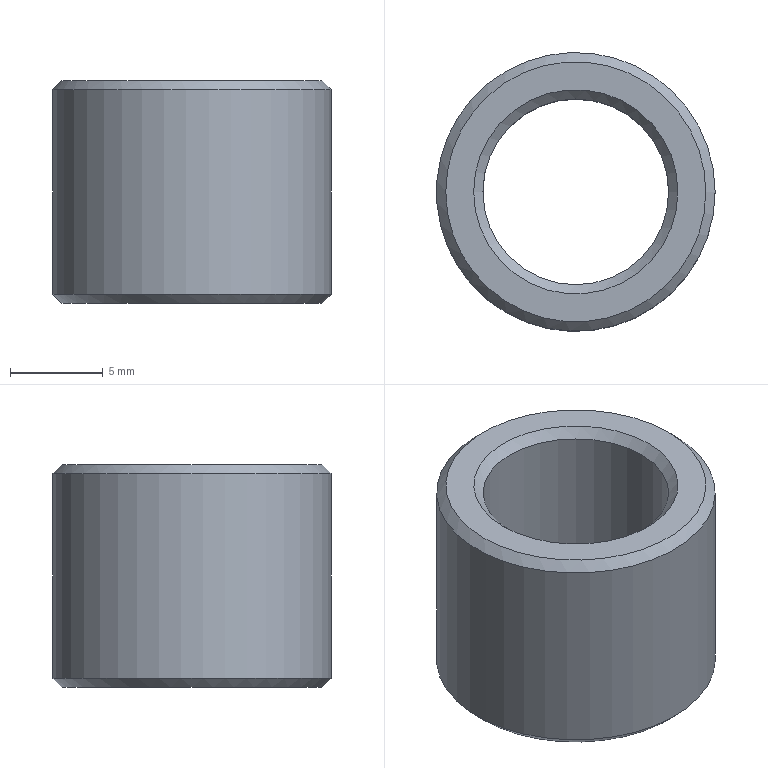Component | NX | BUSHING | 1 solid | 8 faces | box 15 x 15 x 12 mm | volume 1158 mm3 | cone 4 | cylinder 2 | plane 2 | commonest cylinder face diameters 15 x1 10 x1
STEP:
#1=CARTESIAN_POINT('',(0.,0.,0.));
#2=DIRECTION('',(0.,0.,1.));
#3=DIRECTION('',(1.,0.,0.));
#4=AXIS2_PLACEMENT_3D('',#1,#2,#3);
#5=CARTESIAN_POINT('',(19.5,100.638,-216.));
#6=VERTEX_POINT('',#5);
#7=CARTESIAN_POINT('',(12.,100.638,-216.));
#8=DIRECTION('',(0.,0.,1.));
#9=DIRECTION('',(1.,0.,0.));
#10=AXIS2_PLACEMENT_3D('',#7,#8,#9);
#11=CIRCLE('',#10,7.5);
#12=CARTESIAN_POINT('',(12.,100.638,-204.5));
#13=DIRECTION('',(0.,0.,-1.));
#14=DIRECTION('',(-1.,0.,0.));
#15=AXIS2_PLACEMENT_3D('',#12,#13,#14);
#16=CYLINDRICAL_SURFACE('',#15,7.5);
#17=CARTESIAN_POINT('',(9.425,11.5));
#18=DIRECTION('',(-1.,0.));
#19=VECTOR('',#18,1.);
#20=LINE('',#17,#19);
#21=(GEOMETRIC_REPRESENTATION_CONTEXT(2)PARAMETRIC_REPRESENTATION_CONTEXT()REPRESENTATION_CONTEXT('',''));
#22=DEFINITIONAL_REPRESENTATION('',(#20),#21);
#23=PCURVE('',#16,#22);
#24=CARTESIAN_POINT('',(12.,100.638,-216.));
#25=DIRECTION('',(0.,0.,1.));
#26=DIRECTION('',(1.,0.,0.));
#27=AXIS2_PLACEMENT_3D('',#24,#25,#26);
#28=CONICAL_SURFACE('',#27,7.5,0.7854);
#29=CARTESIAN_POINT('',(0.,0.));
#30=DIRECTION('',(1.,0.));
#31=VECTOR('',#30,1.);
#32=LINE('',#29,#31);
#33=(GEOMETRIC_REPRESENTATION_CONTEXT(2)PARAMETRIC_REPRESENTATION_CONTEXT()REPRESENTATION_CONTEXT('',''));
#34=DEFINITIONAL_REPRESENTATION('',(#32),#33);
#35=PCURVE('',#28,#34);
#36=SURFACE_CURVE('',#11,(#23,#35),.PCURVE_S1.);
#37=EDGE_CURVE('',#6,#6,#36,.T.);
#38=ORIENTED_EDGE('',*,*,#37,.T.);
#39=CARTESIAN_POINT('',(19.5,100.638,-205.));
#40=VERTEX_POINT('',#39);
#41=CARTESIAN_POINT('',(19.5,100.638,-205.));
#42=CARTESIAN_POINT('',(19.5,100.638,-216.));
#43=B_SPLINE_CURVE_WITH_KNOTS('',1,(#41,#42),.UNSPECIFIED.,.F.,.F.,(2,2),(0.5,11.5),.PIECEWISE_BEZIER_KNOTS.);
#44=CARTESIAN_POINT('',(3.142,0.));
#45=DIRECTION('',(0.,1.));
#46=VECTOR('',#45,1.);
#47=LINE('',#44,#46);
#48=(GEOMETRIC_REPRESENTATION_CONTEXT(2)PARAMETRIC_REPRESENTATION_CONTEXT()REPRESENTATION_CONTEXT('',''));
#49=DEFINITIONAL_REPRESENTATION('',(#47),#48);
#50=PCURVE('',#16,#49);
#51=CARTESIAN_POINT('',(9.425,0.));
#52=DIRECTION('',(0.,1.));
#53=VECTOR('',#52,1.);
#54=LINE('',#51,#53);
#55=(GEOMETRIC_REPRESENTATION_CONTEXT(2)PARAMETRIC_REPRESENTATION_CONTEXT()REPRESENTATION_CONTEXT('',''));
#56=DEFINITIONAL_REPRESENTATION('',(#54),#55);
#57=PCURVE('',#16,#56);
#58=SEAM_CURVE('',#43,(#50,#57),.PCURVE_S1.);
#59=EDGE_CURVE('',#40,#6,#58,.T.);
#60=ORIENTED_EDGE('',*,*,#59,.F.);
#61=CARTESIAN_POINT('',(12.,100.638,-205.));
#62=DIRECTION('',(0.,0.,-1.));
#63=DIRECTION('',(1.,0.,0.));
#64=AXIS2_PLACEMENT_3D('',#61,#62,#63);
#65=CIRCLE('',#64,7.5);
#66=CARTESIAN_POINT('',(3.142,0.5));
#67=DIRECTION('',(1.,0.));
#68=VECTOR('',#67,1.);
#69=LINE('',#66,#68);
#70=(GEOMETRIC_REPRESENTATION_CONTEXT(2)PARAMETRIC_REPRESENTATION_CONTEXT()REPRESENTATION_CONTEXT('',''));
#71=DEFINITIONAL_REPRESENTATION('',(#69),#70);
#72=PCURVE('',#16,#71);
#73=CARTESIAN_POINT('',(12.,100.638,-204.5));
#74=DIRECTION('',(0.,0.,-1.));
#75=DIRECTION('',(-1.,0.,0.));
#76=AXIS2_PLACEMENT_3D('',#73,#74,#75);
#77=CONICAL_SURFACE('',#76,7.,0.7854);
#78=CARTESIAN_POINT('',(3.142,0.5));
#79=DIRECTION('',(1.,0.));
#80=VECTOR('',#79,1.);
#81=LINE('',#78,#80);
#82=(GEOMETRIC_REPRESENTATION_CONTEXT(2)PARAMETRIC_REPRESENTATION_CONTEXT()REPRESENTATION_CONTEXT('',''));
#83=DEFINITIONAL_REPRESENTATION('',(#81),#82);
#84=PCURVE('',#77,#83);
#85=SURFACE_CURVE('',#65,(#72,#84),.PCURVE_S1.);
#86=EDGE_CURVE('',#40,#40,#85,.T.);
#87=ORIENTED_EDGE('',*,*,#86,.T.);
#88=ORIENTED_EDGE('',*,*,#59,.T.);
#89=EDGE_LOOP('',(#38,#60,#87,#88));
#90=FACE_BOUND('',#89,.T.);
#91=ADVANCED_FACE('',(#90),#16,.T.);
#92=CARTESIAN_POINT('',(17.,100.638,-216.));
#93=VERTEX_POINT('',#92);
#94=CARTESIAN_POINT('',(12.,100.638,-216.));
#95=DIRECTION('',(0.,0.,-1.));
#96=DIRECTION('',(1.,0.,0.));
#97=AXIS2_PLACEMENT_3D('',#94,#95,#96);
#98=CIRCLE('',#97,5.);
#99=CARTESIAN_POINT('',(12.,100.638,-204.5));
#100=DIRECTION('',(0.,0.,-1.));
#101=DIRECTION('',(-1.,0.,0.));
#102=AXIS2_PLACEMENT_3D('',#99,#100,#101);
#103=CYLINDRICAL_SURFACE('',#102,5.);
#104=CARTESIAN_POINT('',(3.142,11.5));
#105=DIRECTION('',(1.,0.));
#106=VECTOR('',#105,1.);
#107=LINE('',#104,#106);
#108=(GEOMETRIC_REPRESENTATION_CONTEXT(2)PARAMETRIC_REPRESENTATION_CONTEXT()REPRESENTATION_CONTEXT('',''));
#109=DEFINITIONAL_REPRESENTATION('',(#107),#108);
#110=PCURVE('',#103,#109);
#111=CARTESIAN_POINT('',(12.,100.638,-216.5));
#112=DIRECTION('',(0.,0.,-1.));
#113=DIRECTION('',(-1.,0.,0.));
#114=AXIS2_PLACEMENT_3D('',#111,#112,#113);
#115=CONICAL_SURFACE('',#114,5.5,0.7854);
#116=CARTESIAN_POINT('',(3.142,-0.5));
#117=DIRECTION('',(1.,0.));
#118=VECTOR('',#117,1.);
#119=LINE('',#116,#118);
#120=(GEOMETRIC_REPRESENTATION_CONTEXT(2)PARAMETRIC_REPRESENTATION_CONTEXT()REPRESENTATION_CONTEXT('',''));
#121=DEFINITIONAL_REPRESENTATION('',(#119),#120);
#122=PCURVE('',#115,#121);
#123=SURFACE_CURVE('',#98,(#110,#122),.PCURVE_S1.);
#124=EDGE_CURVE('',#93,#93,#123,.T.);
#125=ORIENTED_EDGE('',*,*,#124,.F.);
#126=CARTESIAN_POINT('',(17.,100.638,-205.));
#127=VERTEX_POINT('',#126);
#128=CARTESIAN_POINT('',(17.,100.638,-205.));
#129=CARTESIAN_POINT('',(17.,100.638,-216.));
#130=B_SPLINE_CURVE_WITH_KNOTS('',1,(#128,#129),.UNSPECIFIED.,.F.,.F.,(2,2),(0.5,11.5),.PIECEWISE_BEZIER_KNOTS.);
#131=CARTESIAN_POINT('',(3.142,0.));
#132=DIRECTION('',(0.,1.));
#133=VECTOR('',#132,1.);
#134=LINE('',#131,#133);
#135=(GEOMETRIC_REPRESENTATION_CONTEXT(2)PARAMETRIC_REPRESENTATION_CONTEXT()REPRESENTATION_CONTEXT('',''));
#136=DEFINITIONAL_REPRESENTATION('',(#134),#135);
#137=PCURVE('',#103,#136);
#138=CARTESIAN_POINT('',(9.425,0.));
#139=DIRECTION('',(0.,1.));
#140=VECTOR('',#139,1.);
#141=LINE('',#138,#140);
#142=(GEOMETRIC_REPRESENTATION_CONTEXT(2)PARAMETRIC_REPRESENTATION_CONTEXT()REPRESENTATION_CONTEXT('',''));
#143=DEFINITIONAL_REPRESENTATION('',(#141),#142);
#144=PCURVE('',#103,#143);
#145=SEAM_CURVE('',#130,(#137,#144),.PCURVE_S1.);
#146=EDGE_CURVE('',#127,#93,#145,.T.);
#147=ORIENTED_EDGE('',*,*,#146,.F.);
#148=CARTESIAN_POINT('',(12.,100.638,-205.));
#149=DIRECTION('',(0.,0.,1.));
#150=DIRECTION('',(1.,0.,0.));
#151=AXIS2_PLACEMENT_3D('',#148,#149,#150);
#152=CIRCLE('',#151,5.);
#153=CARTESIAN_POINT('',(9.425,0.5));
#154=DIRECTION('',(-1.,0.));
#155=VECTOR('',#154,1.);
#156=LINE('',#153,#155);
#157=(GEOMETRIC_REPRESENTATION_CONTEXT(2)PARAMETRIC_REPRESENTATION_CONTEXT()REPRESENTATION_CONTEXT('',''));
#158=DEFINITIONAL_REPRESENTATION('',(#156),#157);
#159=PCURVE('',#103,#158);
#160=CARTESIAN_POINT('',(12.,100.638,-205.));
#161=DIRECTION('',(0.,0.,1.));
#162=DIRECTION('',(1.,0.,0.));
#163=AXIS2_PLACEMENT_3D('',#160,#161,#162);
#164=CONICAL_SURFACE('',#163,5.,0.7854);
#165=CARTESIAN_POINT('',(0.,0.));
#166=DIRECTION('',(1.,0.));
#167=VECTOR('',#166,1.);
#168=LINE('',#165,#167);
#169=(GEOMETRIC_REPRESENTATION_CONTEXT(2)PARAMETRIC_REPRESENTATION_CONTEXT()REPRESENTATION_CONTEXT('',''));
#170=DEFINITIONAL_REPRESENTATION('',(#168),#169);
#171=PCURVE('',#164,#170);
#172=SURFACE_CURVE('',#152,(#159,#171),.PCURVE_S1.);
#173=EDGE_CURVE('',#127,#127,#172,.T.);
#174=ORIENTED_EDGE('',*,*,#173,.F.);
#175=ORIENTED_EDGE('',*,*,#146,.T.);
#176=EDGE_LOOP('',(#125,#147,#174,#175));
#177=FACE_BOUND('',#176,.F.);
#178=ADVANCED_FACE('',(#177),#103,.F.);
#179=CARTESIAN_POINT('',(17.5,100.638,-204.5));
#180=VERTEX_POINT('',#179);
#181=CARTESIAN_POINT('',(12.,100.638,-204.5));
#182=DIRECTION('',(0.,0.,-1.));
#183=DIRECTION('',(1.,0.,0.));
#184=AXIS2_PLACEMENT_3D('',#181,#182,#183);
#185=CIRCLE('',#184,5.5);
#186=CARTESIAN_POINT('',(12.,100.638,-204.5));
#187=DIRECTION('',(0.,0.,1.));
#188=DIRECTION('',(1.,0.,0.));
#189=AXIS2_PLACEMENT_3D('',#186,#187,#188);
#190=PLANE('',#189);
#191=CARTESIAN_POINT('',(5.5,0.));
#192=CARTESIAN_POINT('',(5.5,-9.526));
#193=CARTESIAN_POINT('',(-2.75,-4.763));
#194=CARTESIAN_POINT('',(-11.,-0.));
#195=CARTESIAN_POINT('',(-2.75,4.763));
#196=CARTESIAN_POINT('',(5.5,9.526));
#197=CARTESIAN_POINT('',(5.5,0.));
#198=(BOUNDED_CURVE()B_SPLINE_CURVE(2,(#191,#192,#193,#194,#195,#196,#197),.UNSPECIFIED.,.T.,.F.)B_SPLINE_CURVE_WITH_KNOTS((1,2,2,2,2,1),(-2.094,0.,2.094,4.189,6.283,8.378),.UNSPECIFIED.)CURVE()GEOMETRIC_REPRESENTATION_ITEM()RATIONAL_B_SPLINE_CURVE((1.,0.5,1.,0.5,1.,0.5,1.))REPRESENTATION_ITEM(''));
#199=(GEOMETRIC_REPRESENTATION_CONTEXT(2)PARAMETRIC_REPRESENTATION_CONTEXT()REPRESENTATION_CONTEXT('',''));
#200=DEFINITIONAL_REPRESENTATION('',(#198),#199);
#201=PCURVE('',#190,#200);
#202=CARTESIAN_POINT('',(6.283,0.5));
#203=DIRECTION('',(-1.,0.));
#204=VECTOR('',#203,1.);
#205=LINE('',#202,#204);
#206=(GEOMETRIC_REPRESENTATION_CONTEXT(2)PARAMETRIC_REPRESENTATION_CONTEXT()REPRESENTATION_CONTEXT('',''));
#207=DEFINITIONAL_REPRESENTATION('',(#205),#206);
#208=PCURVE('',#164,#207);
#209=SURFACE_CURVE('',#185,(#201,#208),.PCURVE_S1.);
#210=EDGE_CURVE('',#180,#180,#209,.T.);
#211=ORIENTED_EDGE('',*,*,#210,.T.);
#212=EDGE_LOOP('',(#211));
#213=FACE_BOUND('',#212,.T.);
#214=CARTESIAN_POINT('',(19.,100.638,-204.5));
#215=VERTEX_POINT('',#214);
#216=CARTESIAN_POINT('',(12.,100.638,-204.5));
#217=DIRECTION('',(0.,0.,1.));
#218=DIRECTION('',(1.,0.,0.));
#219=AXIS2_PLACEMENT_3D('',#216,#217,#218);
#220=CIRCLE('',#219,7.);
#221=CARTESIAN_POINT('',(0.,0.));
#222=DIRECTION('',(1.,0.));
#223=AXIS2_PLACEMENT_2D('',#221,#222);
#224=CIRCLE('',#223,7.);
#225=(GEOMETRIC_REPRESENTATION_CONTEXT(2)PARAMETRIC_REPRESENTATION_CONTEXT()REPRESENTATION_CONTEXT('',''));
#226=DEFINITIONAL_REPRESENTATION('',(#224),#225);
#227=PCURVE('',#190,#226);
#228=CARTESIAN_POINT('',(9.425,0.));
#229=DIRECTION('',(-1.,0.));
#230=VECTOR('',#229,1.);
#231=LINE('',#228,#230);
#232=(GEOMETRIC_REPRESENTATION_CONTEXT(2)PARAMETRIC_REPRESENTATION_CONTEXT()REPRESENTATION_CONTEXT('',''));
#233=DEFINITIONAL_REPRESENTATION('',(#231),#232);
#234=PCURVE('',#77,#233);
#235=SURFACE_CURVE('',#220,(#227,#234),.PCURVE_S1.);
#236=EDGE_CURVE('',#215,#215,#235,.T.);
#237=ORIENTED_EDGE('',*,*,#236,.T.);
#238=EDGE_LOOP('',(#237));
#239=FACE_BOUND('',#238,.T.);
#240=ADVANCED_FACE('',(#213,#239),#190,.T.);
#241=CARTESIAN_POINT('',(17.5,100.638,-216.5));
#242=VERTEX_POINT('',#241);
#243=CARTESIAN_POINT('',(12.,100.638,-216.5));
#244=DIRECTION('',(0.,0.,1.));
#245=DIRECTION('',(1.,0.,0.));
#246=AXIS2_PLACEMENT_3D('',#243,#244,#245);
#247=CIRCLE('',#246,5.5);
#248=CARTESIAN_POINT('',(12.,100.638,-216.5));
#249=DIRECTION('',(0.,0.,1.));
#250=DIRECTION('',(1.,0.,0.));
#251=AXIS2_PLACEMENT_3D('',#248,#249,#250);
#252=PLANE('',#251);
#253=CARTESIAN_POINT('',(0.,0.));
#254=DIRECTION('',(1.,0.));
#255=AXIS2_PLACEMENT_2D('',#253,#254);
#256=CIRCLE('',#255,5.5);
#257=(GEOMETRIC_REPRESENTATION_CONTEXT(2)PARAMETRIC_REPRESENTATION_CONTEXT()REPRESENTATION_CONTEXT('',''));
#258=DEFINITIONAL_REPRESENTATION('',(#256),#257);
#259=PCURVE('',#252,#258);
#260=CARTESIAN_POINT('',(9.425,0.));
#261=DIRECTION('',(-1.,0.));
#262=VECTOR('',#261,1.);
#263=LINE('',#260,#262);
#264=(GEOMETRIC_REPRESENTATION_CONTEXT(2)PARAMETRIC_REPRESENTATION_CONTEXT()REPRESENTATION_CONTEXT('',''));
#265=DEFINITIONAL_REPRESENTATION('',(#263),#264);
#266=PCURVE('',#115,#265);
#267=SURFACE_CURVE('',#247,(#259,#266),.PCURVE_S1.);
#268=EDGE_CURVE('',#242,#242,#267,.T.);
#269=ORIENTED_EDGE('',*,*,#268,.T.);
#270=EDGE_LOOP('',(#269));
#271=FACE_BOUND('',#270,.T.);
#272=CARTESIAN_POINT('',(19.,100.638,-216.5));
#273=VERTEX_POINT('',#272);
#274=CARTESIAN_POINT('',(12.,100.638,-216.5));
#275=DIRECTION('',(0.,0.,-1.));
#276=DIRECTION('',(1.,0.,0.));
#277=AXIS2_PLACEMENT_3D('',#274,#275,#276);
#278=CIRCLE('',#277,7.);
#279=CARTESIAN_POINT('',(7.,0.));
#280=CARTESIAN_POINT('',(7.,-12.124));
#281=CARTESIAN_POINT('',(-3.5,-6.062));
#282=CARTESIAN_POINT('',(-14.,-0.));
#283=CARTESIAN_POINT('',(-3.5,6.062));
#284=CARTESIAN_POINT('',(7.,12.124));
#285=CARTESIAN_POINT('',(7.,0.));
#286=(BOUNDED_CURVE()B_SPLINE_CURVE(2,(#279,#280,#281,#282,#283,#284,#285),.UNSPECIFIED.,.T.,.F.)B_SPLINE_CURVE_WITH_KNOTS((1,2,2,2,2,1),(-2.094,0.,2.094,4.189,6.283,8.378),.UNSPECIFIED.)CURVE()GEOMETRIC_REPRESENTATION_ITEM()RATIONAL_B_SPLINE_CURVE((1.,0.5,1.,0.5,1.,0.5,1.))REPRESENTATION_ITEM(''));
#287=(GEOMETRIC_REPRESENTATION_CONTEXT(2)PARAMETRIC_REPRESENTATION_CONTEXT()REPRESENTATION_CONTEXT('',''));
#288=DEFINITIONAL_REPRESENTATION('',(#286),#287);
#289=PCURVE('',#252,#288);
#290=CARTESIAN_POINT('',(6.283,-0.5));
#291=DIRECTION('',(-1.,0.));
#292=VECTOR('',#291,1.);
#293=LINE('',#290,#292);
#294=(GEOMETRIC_REPRESENTATION_CONTEXT(2)PARAMETRIC_REPRESENTATION_CONTEXT()REPRESENTATION_CONTEXT('',''));
#295=DEFINITIONAL_REPRESENTATION('',(#293),#294);
#296=PCURVE('',#28,#295);
#297=SURFACE_CURVE('',#278,(#289,#296),.PCURVE_S1.);
#298=EDGE_CURVE('',#273,#273,#297,.T.);
#299=ORIENTED_EDGE('',*,*,#298,.T.);
#300=EDGE_LOOP('',(#299));
#301=FACE_BOUND('',#300,.T.);
#302=ADVANCED_FACE('',(#271,#301),#252,.F.);
#303=ORIENTED_EDGE('',*,*,#124,.T.);
#304=CARTESIAN_POINT('',(17.,100.638,-216.));
#305=CARTESIAN_POINT('',(17.5,100.638,-216.5));
#306=B_SPLINE_CURVE_WITH_KNOTS('',1,(#304,#305),.UNSPECIFIED.,.F.,.F.,(2,2),(-0.7071,0.),.PIECEWISE_BEZIER_KNOTS.);
#307=CARTESIAN_POINT('',(9.425,0.));
#308=DIRECTION('',(0.,1.));
#309=VECTOR('',#308,1.);
#310=LINE('',#307,#309);
#311=(GEOMETRIC_REPRESENTATION_CONTEXT(2)PARAMETRIC_REPRESENTATION_CONTEXT()REPRESENTATION_CONTEXT('',''));
#312=DEFINITIONAL_REPRESENTATION('',(#310),#311);
#313=PCURVE('',#115,#312);
#314=CARTESIAN_POINT('',(3.142,0.));
#315=DIRECTION('',(0.,1.));
#316=VECTOR('',#315,1.);
#317=LINE('',#314,#316);
#318=(GEOMETRIC_REPRESENTATION_CONTEXT(2)PARAMETRIC_REPRESENTATION_CONTEXT()REPRESENTATION_CONTEXT('',''));
#319=DEFINITIONAL_REPRESENTATION('',(#317),#318);
#320=PCURVE('',#115,#319);
#321=SEAM_CURVE('',#306,(#313,#320),.PCURVE_S1.);
#322=EDGE_CURVE('',#93,#242,#321,.T.);
#323=ORIENTED_EDGE('',*,*,#322,.T.);
#324=ORIENTED_EDGE('',*,*,#268,.T.);
#325=ORIENTED_EDGE('',*,*,#322,.F.);
#326=EDGE_LOOP('',(#303,#323,#324,#325));
#327=FACE_BOUND('',#326,.F.);
#328=ADVANCED_FACE('',(#327),#115,.F.);
#329=ORIENTED_EDGE('',*,*,#298,.F.);
#330=CARTESIAN_POINT('',(19.,100.638,-216.5));
#331=CARTESIAN_POINT('',(19.5,100.638,-216.));
#332=B_SPLINE_CURVE_WITH_KNOTS('',1,(#330,#331),.UNSPECIFIED.,.F.,.F.,(2,2),(-0.7071,0.),.PIECEWISE_BEZIER_KNOTS.);
#333=CARTESIAN_POINT('',(6.283,0.));
#334=DIRECTION('',(0.,1.));
#335=VECTOR('',#334,1.);
#336=LINE('',#333,#335);
#337=(GEOMETRIC_REPRESENTATION_CONTEXT(2)PARAMETRIC_REPRESENTATION_CONTEXT()REPRESENTATION_CONTEXT('',''));
#338=DEFINITIONAL_REPRESENTATION('',(#336),#337);
#339=PCURVE('',#28,#338);
#340=CARTESIAN_POINT('',(0.,0.));
#341=DIRECTION('',(0.,1.));
#342=VECTOR('',#341,1.);
#343=LINE('',#340,#342);
#344=(GEOMETRIC_REPRESENTATION_CONTEXT(2)PARAMETRIC_REPRESENTATION_CONTEXT()REPRESENTATION_CONTEXT('',''));
#345=DEFINITIONAL_REPRESENTATION('',(#343),#344);
#346=PCURVE('',#28,#345);
#347=SEAM_CURVE('',#332,(#339,#346),.PCURVE_S1.);
#348=EDGE_CURVE('',#273,#6,#347,.T.);
#349=ORIENTED_EDGE('',*,*,#348,.T.);
#350=ORIENTED_EDGE('',*,*,#37,.F.);
#351=ORIENTED_EDGE('',*,*,#348,.F.);
#352=EDGE_LOOP('',(#329,#349,#350,#351));
#353=FACE_BOUND('',#352,.T.);
#354=ADVANCED_FACE('',(#353),#28,.T.);
#355=ORIENTED_EDGE('',*,*,#210,.T.);
#356=CARTESIAN_POINT('',(17.,100.638,-205.));
#357=CARTESIAN_POINT('',(17.5,100.638,-204.5));
#358=B_SPLINE_CURVE_WITH_KNOTS('',1,(#356,#357),.UNSPECIFIED.,.F.,.F.,(2,2),(0.,0.7071),.PIECEWISE_BEZIER_KNOTS.);
#359=CARTESIAN_POINT('',(0.,0.));
#360=DIRECTION('',(0.,1.));
#361=VECTOR('',#360,1.);
#362=LINE('',#359,#361);
#363=(GEOMETRIC_REPRESENTATION_CONTEXT(2)PARAMETRIC_REPRESENTATION_CONTEXT()REPRESENTATION_CONTEXT('',''));
#364=DEFINITIONAL_REPRESENTATION('',(#362),#363);
#365=PCURVE('',#164,#364);
#366=CARTESIAN_POINT('',(6.283,0.));
#367=DIRECTION('',(0.,1.));
#368=VECTOR('',#367,1.);
#369=LINE('',#366,#368);
#370=(GEOMETRIC_REPRESENTATION_CONTEXT(2)PARAMETRIC_REPRESENTATION_CONTEXT()REPRESENTATION_CONTEXT('',''));
#371=DEFINITIONAL_REPRESENTATION('',(#369),#370);
#372=PCURVE('',#164,#371);
#373=SEAM_CURVE('',#358,(#365,#372),.PCURVE_S1.);
#374=EDGE_CURVE('',#127,#180,#373,.T.);
#375=ORIENTED_EDGE('',*,*,#374,.F.);
#376=ORIENTED_EDGE('',*,*,#173,.T.);
#377=ORIENTED_EDGE('',*,*,#374,.T.);
#378=EDGE_LOOP('',(#355,#375,#376,#377));
#379=FACE_BOUND('',#378,.F.);
#380=ADVANCED_FACE('',(#379),#164,.F.);
#381=ORIENTED_EDGE('',*,*,#86,.F.);
#382=CARTESIAN_POINT('',(19.,100.638,-204.5));
#383=CARTESIAN_POINT('',(19.5,100.638,-205.));
#384=B_SPLINE_CURVE_WITH_KNOTS('',1,(#382,#383),.UNSPECIFIED.,.F.,.F.,(2,2),(0.,0.7071),.PIECEWISE_BEZIER_KNOTS.);
#385=CARTESIAN_POINT('',(3.142,0.));
#386=DIRECTION('',(0.,1.));
#387=VECTOR('',#386,1.);
#388=LINE('',#385,#387);
#389=(GEOMETRIC_REPRESENTATION_CONTEXT(2)PARAMETRIC_REPRESENTATION_CONTEXT()REPRESENTATION_CONTEXT('',''));
#390=DEFINITIONAL_REPRESENTATION('',(#388),#389);
#391=PCURVE('',#77,#390);
#392=CARTESIAN_POINT('',(9.425,0.));
#393=DIRECTION('',(0.,1.));
#394=VECTOR('',#393,1.);
#395=LINE('',#392,#394);
#396=(GEOMETRIC_REPRESENTATION_CONTEXT(2)PARAMETRIC_REPRESENTATION_CONTEXT()REPRESENTATION_CONTEXT('',''));
#397=DEFINITIONAL_REPRESENTATION('',(#395),#396);
#398=PCURVE('',#77,#397);
#399=SEAM_CURVE('',#384,(#391,#398),.PCURVE_S1.);
#400=EDGE_CURVE('',#215,#40,#399,.T.);
#401=ORIENTED_EDGE('',*,*,#400,.F.);
#402=ORIENTED_EDGE('',*,*,#236,.F.);
#403=ORIENTED_EDGE('',*,*,#400,.T.);
#404=EDGE_LOOP('',(#381,#401,#402,#403));
#405=FACE_BOUND('',#404,.T.);
#406=ADVANCED_FACE('',(#405),#77,.T.);
#407=CLOSED_SHELL('',(#91,#178,#240,#302,#328,#354,#380,#406));
#408=MANIFOLD_SOLID_BREP('',#407);
#409=(LENGTH_UNIT()NAMED_UNIT(*)SI_UNIT(.MILLI.,.METRE.));
#410=UNCERTAINTY_MEASURE_WITH_UNIT(LENGTH_MEASURE(0.00001),#409,'','');
#411=(NAMED_UNIT(*)PLANE_ANGLE_UNIT()SI_UNIT($,.RADIAN.));
#412=(NAMED_UNIT(*)SI_UNIT($,.STERADIAN.)SOLID_ANGLE_UNIT());
#413=(GEOMETRIC_REPRESENTATION_CONTEXT(3)GLOBAL_UNCERTAINTY_ASSIGNED_CONTEXT((#410))GLOBAL_UNIT_ASSIGNED_CONTEXT((#409,#411,#412))REPRESENTATION_CONTEXT('',''));
#414=ADVANCED_BREP_SHAPE_REPRESENTATION('',(#4,#408),#413);